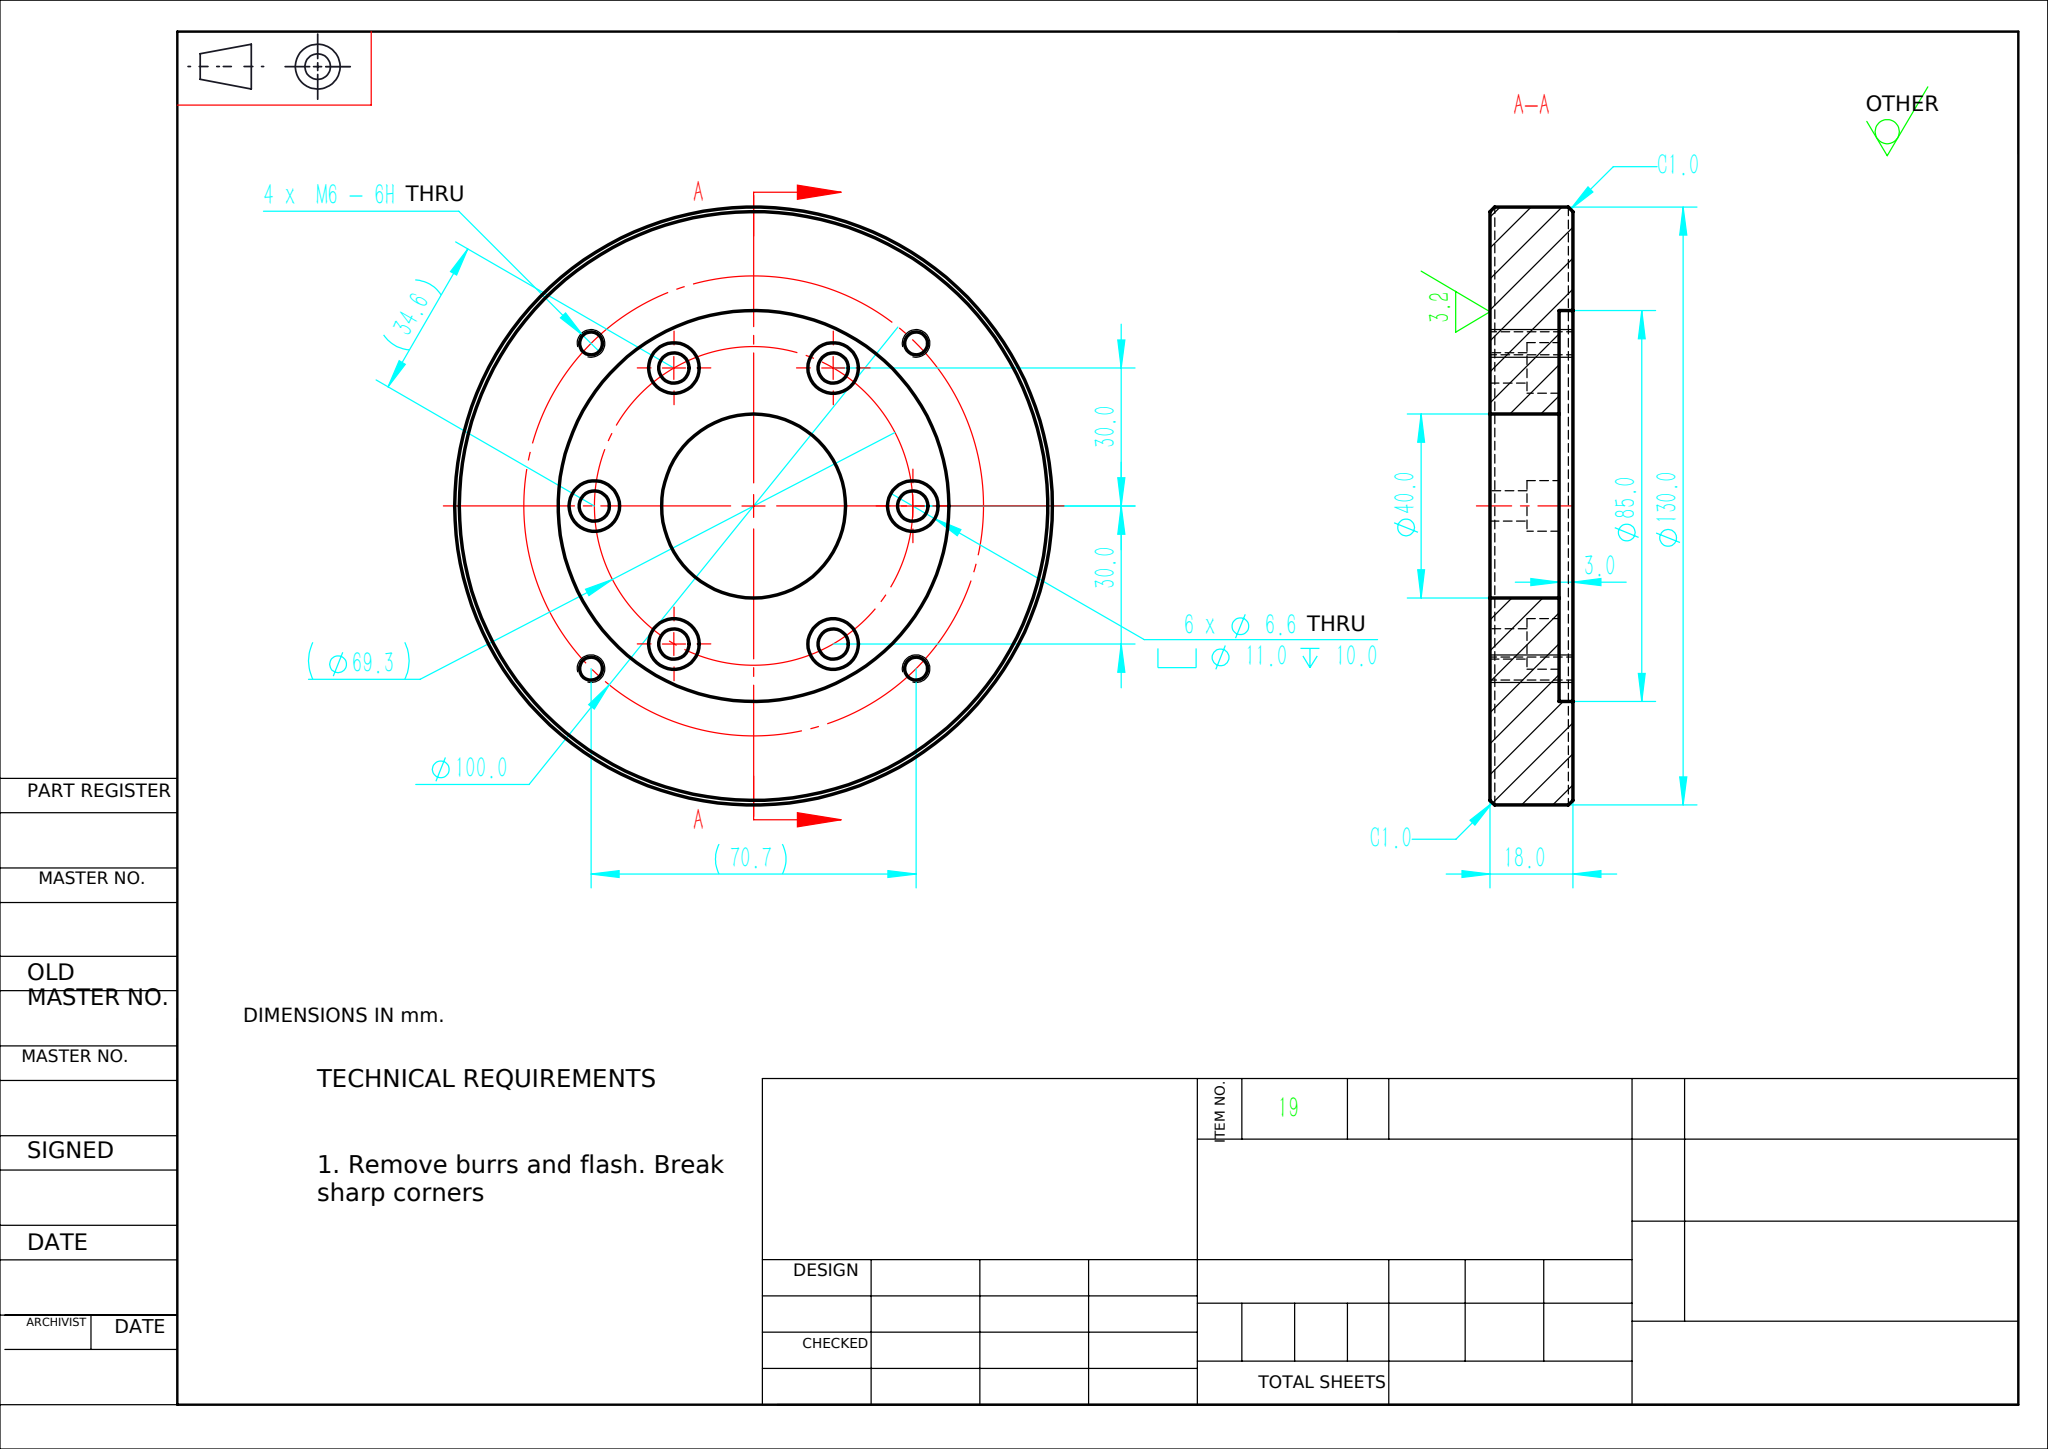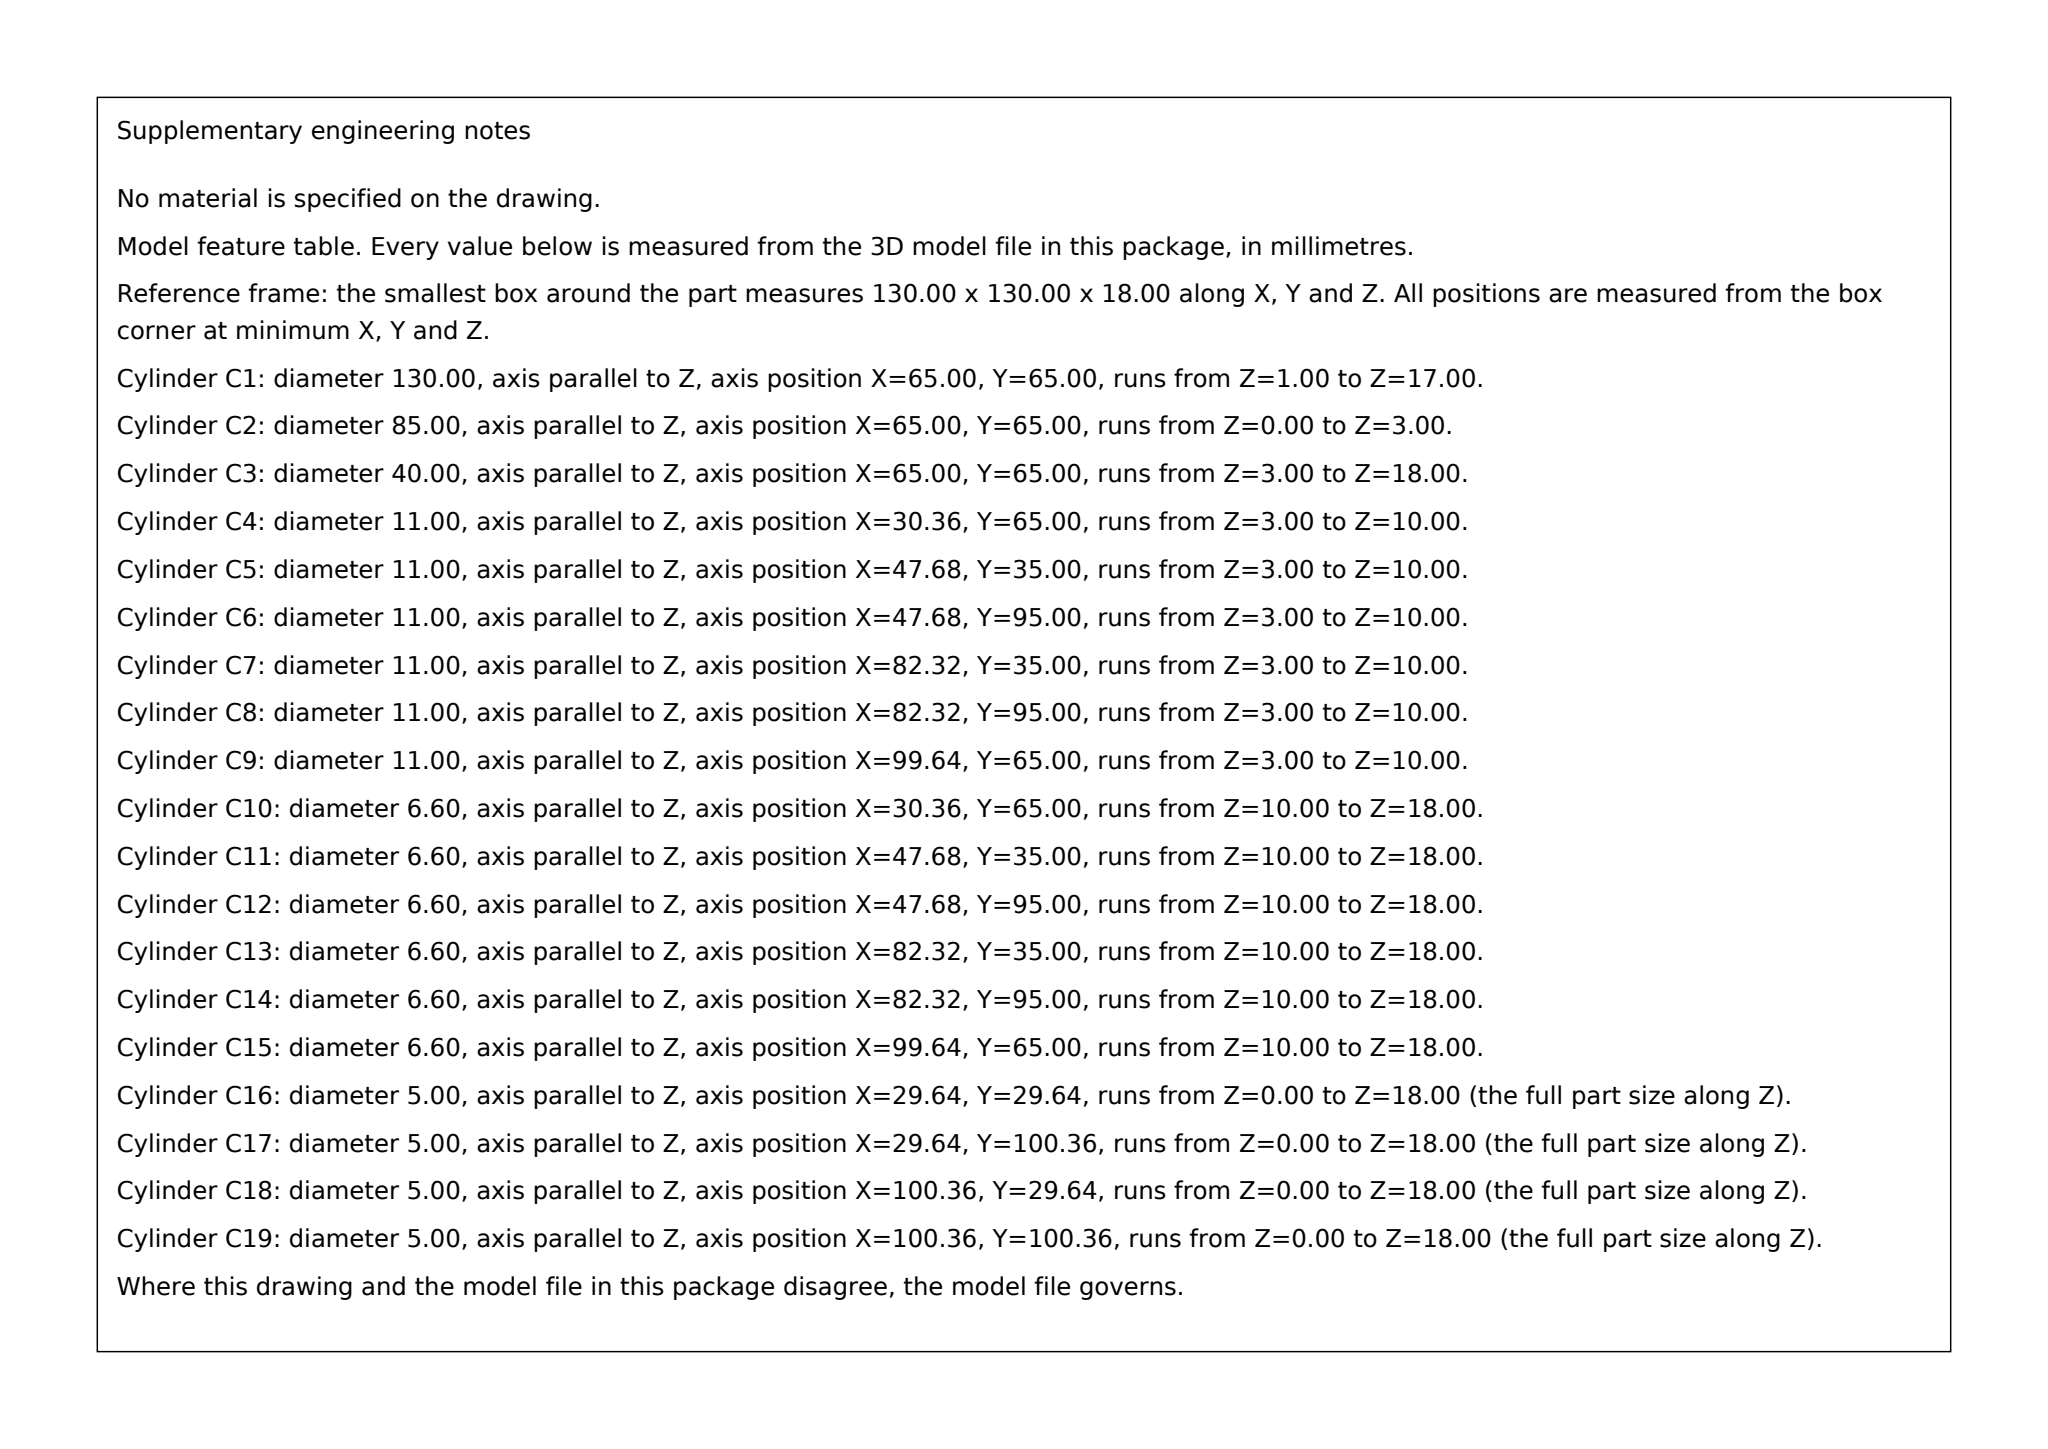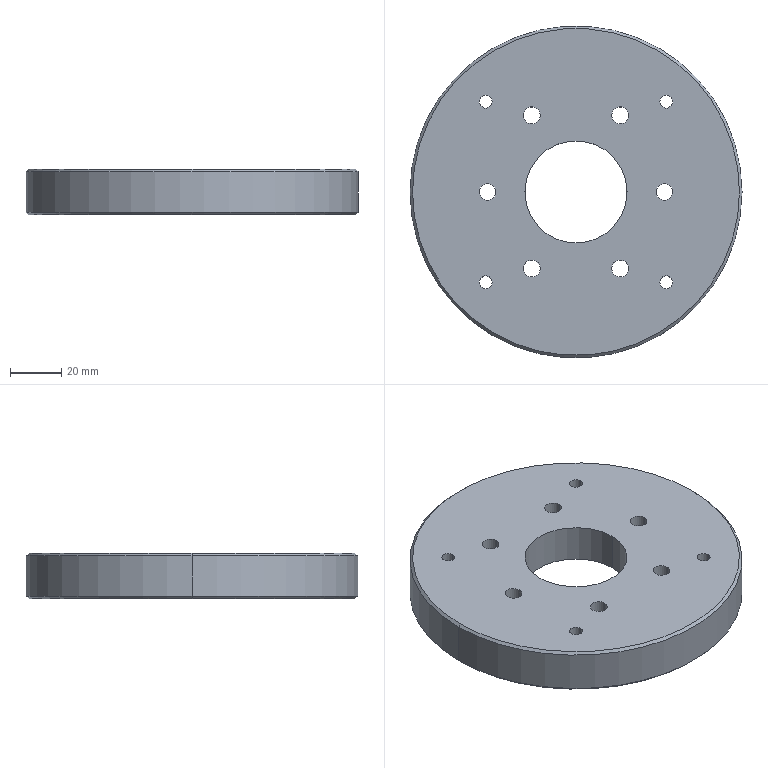Part | SolidWorks | mm | 1 solid | 51 faces | box 130 x 130 x 18 mm | volume 195591 mm3 | cylinder 38 | plane 9 | cone 4 | commonest cylinder face diameters 6.6 x12 11 x12 5 x8 85 x2 130 x2 40 x2
build123d program:
from build123d import *

# Parameters (mm, degrees)
SKETCH1_R                                         = 65
BOSS_EXTRUDE1_DEPTH                               = 18
HOLE_SIZE_ACCORDING_TO_TYPE_0_OF_HEXA_D           = 6.6
HOLE_SIZE_ACCORDING_TO_TYPE_0_OF_HEXA_CBORE_D     = 11
HOLE_SIZE_ACCORDING_TO_TYPE_0_OF_HEXA_CBORE_DEPTH = 10
CHAMFER1_SIZE                                     = 1
M6_TAPPED_HOLE1_D                                 = 5
SKETCH8_R                                         = 42.5
CUT_EXTRUDE1_DEPTH                                = 3


with BuildPart() as part:
    # Sketch1 → Boss-Extrude1 (new body)
    with BuildSketch(Plane.XY):
        Circle(SKETCH1_R)
    extrude(amount=BOSS_EXTRUDE1_DEPTH)

    # Hole Size _ according to_ Type 0 of Hexa (through all)
    with Locations(Plane(origin=(0, 0, 0), x_dir=(-1, 0, 0), z_dir=(0, 0, -1))):
        with Locations((34.641, 0), (-17.321, -30), (-17.321, 30), (17.321, 30), (17.321, -30), (-34.641, 0)):
            CounterBoreHole(HOLE_SIZE_ACCORDING_TO_TYPE_0_OF_HEXA_D / 2, HOLE_SIZE_ACCORDING_TO_TYPE_0_OF_HEXA_CBORE_D / 2, HOLE_SIZE_ACCORDING_TO_TYPE_0_OF_HEXA_CBORE_DEPTH)

    # Sketch4 → Cut-Revolve1 (revolve, cut)
    with BuildSketch(Plane(origin=(0, 0, 0), x_dir=(1, 0, 0), z_dir=(0, 1, 0)), mode=Mode.PRIVATE) as cut_revolve1_sk:
        Polygon((0, -3), (0, -18), (20, -18), (20, 0), (0, 0), align=None)
    revolve(cut_revolve1_sk.sketch.rotate(Axis((0, 0, 3), (0, 0, 1)), 180), axis=Axis((0, 0, 3), (0, 0, 1)), mode=Mode.SUBTRACT)

    # Chamfer1
    chamfer1_edges = [part.edges().sort_by_distance(p)[0] for p in [
        (-65, 0, 0),
        (-65, 0, 18),
    ]]
    chamfer(chamfer1_edges, length=CHAMFER1_SIZE)

    # M6 Tapped Hole1 (through all)
    with Locations(Plane(origin=(0, 0, 0), x_dir=(-1, 0, 0), z_dir=(0, 0, -1))):
        with Locations((35.355, 35.355), (-35.355, 35.355), (-35.355, -35.355), (35.355, -35.355)):
            Hole(M6_TAPPED_HOLE1_D / 2)

    # Sketch8 → Cut-Extrude1 (cut)
    with BuildSketch(Plane(origin=(0, 0, 0), x_dir=(-1, 0, 0), z_dir=(0, 0, -1))):
        Circle(SKETCH8_R)
    extrude(amount=-CUT_EXTRUDE1_DEPTH, mode=Mode.SUBTRACT)


solid = part.part